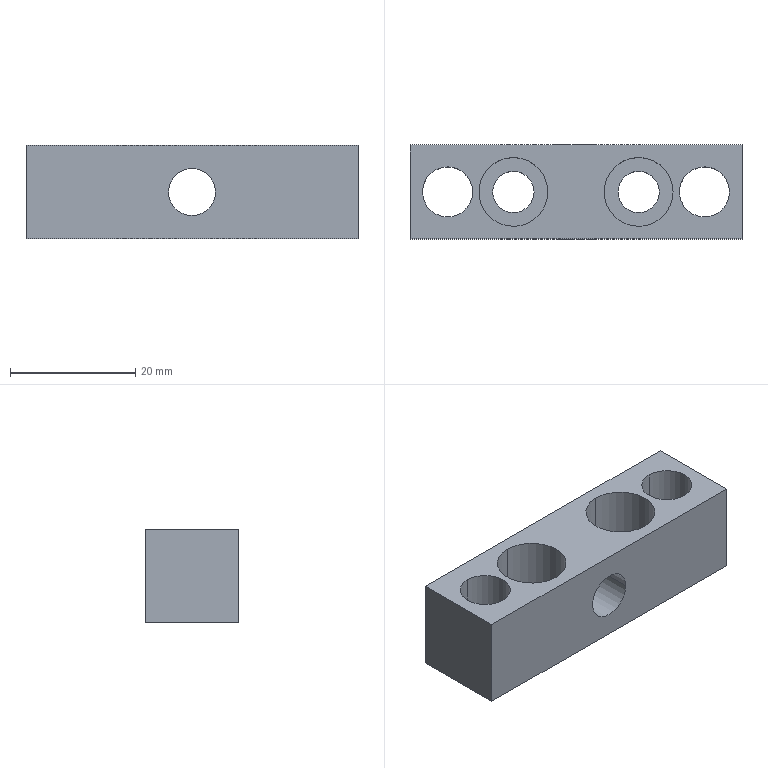CAM job | Mastercam | mm | 17 operations | part box 53 x 15 x 15
1. Facing | 13 - 50 圆鼻铣刀
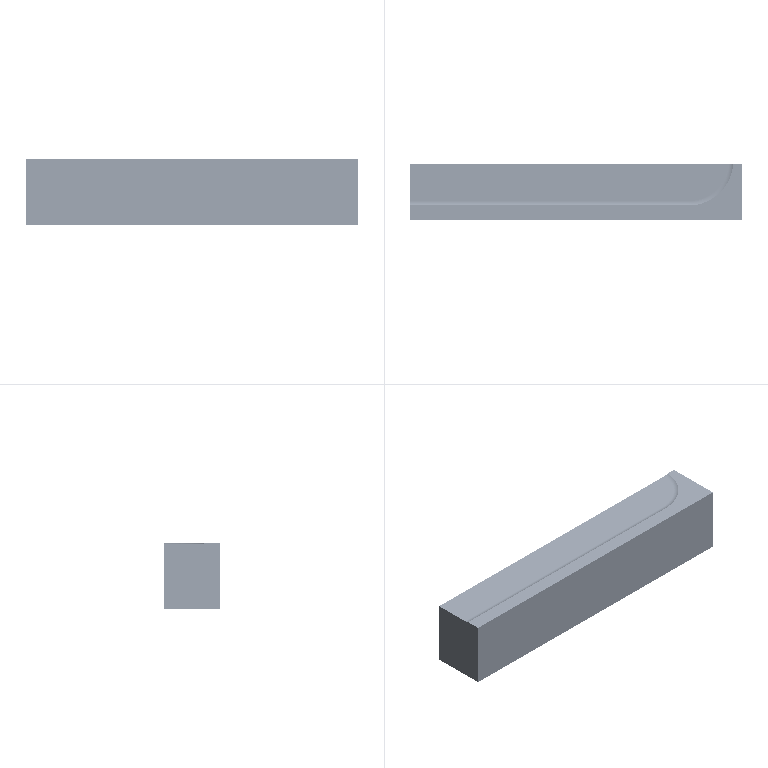2. Peck Drill | 19 - 5 钻头
3. Contour (Ramp) | 4 - 6 平铣刀
4. Contour (Ramp) | 4 - 6 平铣刀
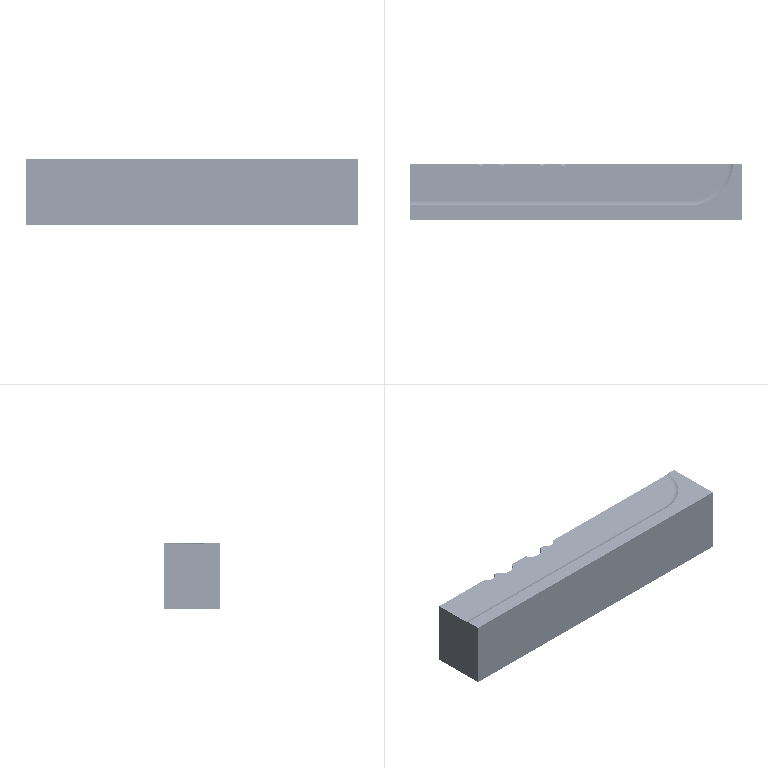5. Contour (Ramp) | 4 - 6 平铣刀
6. Contour (2D) | 5 - 6 平铣刀
7. Contour (2D) | 5 - 6 平铣刀
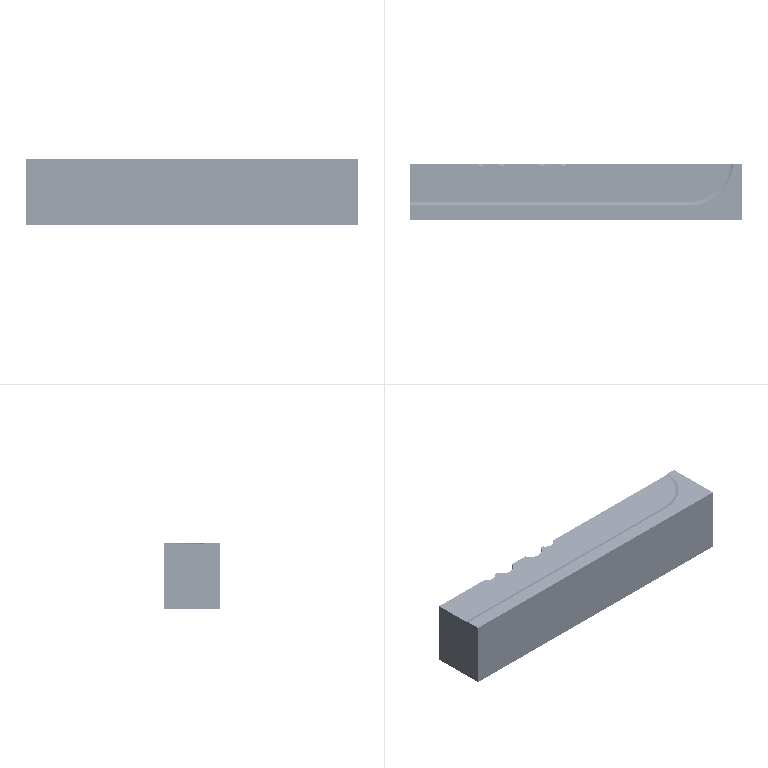8. Contour (2D) | 5 - 6 平铣刀
9. Contour (2D) | 2 - 12 平铣刀
10. Contour (2D) | 3 - 12 平铣刀
11. Model Chamfer | 6 - 6 倒角刀
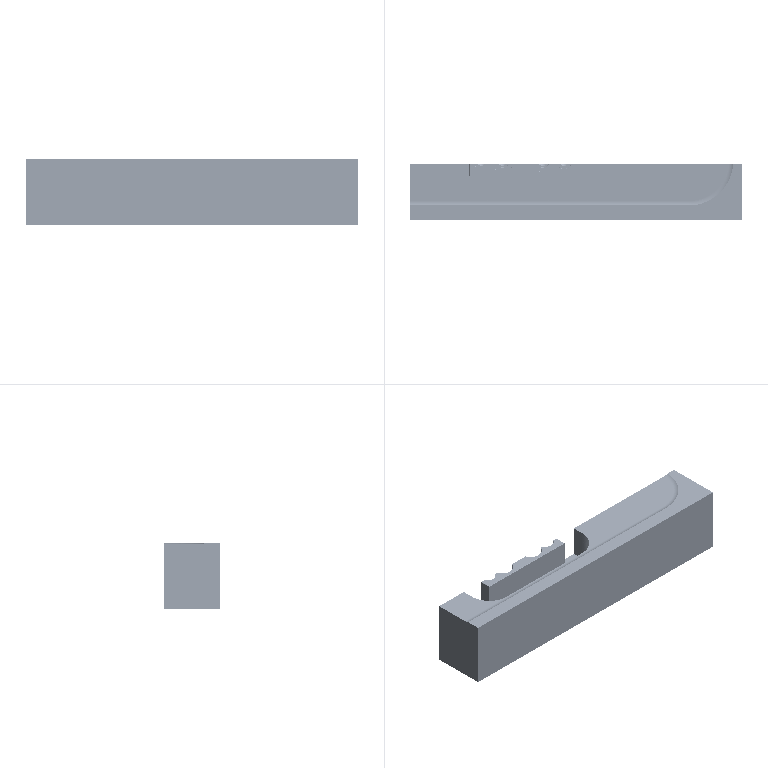12. Facing | 13 - 50 圆鼻铣刀
13. Facing | 13 - 50 圆鼻铣刀
14. Model Chamfer | 6 - 6 倒角刀
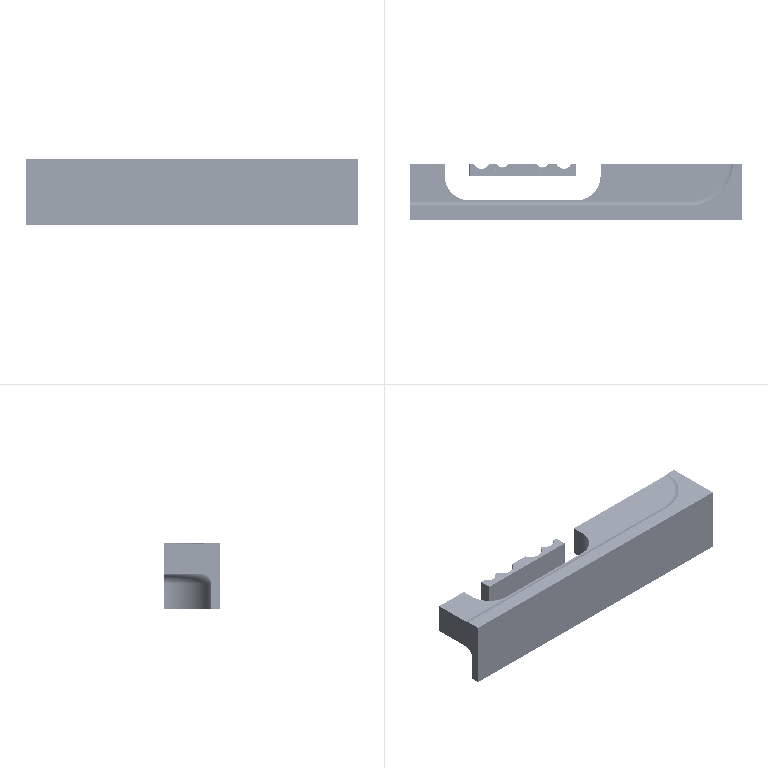15. Contour (Ramp) | 4 - 6 平铣刀
16. Contour (2D) | 5 - 6 平铣刀
17. Model Chamfer | 6 - 6 倒角刀